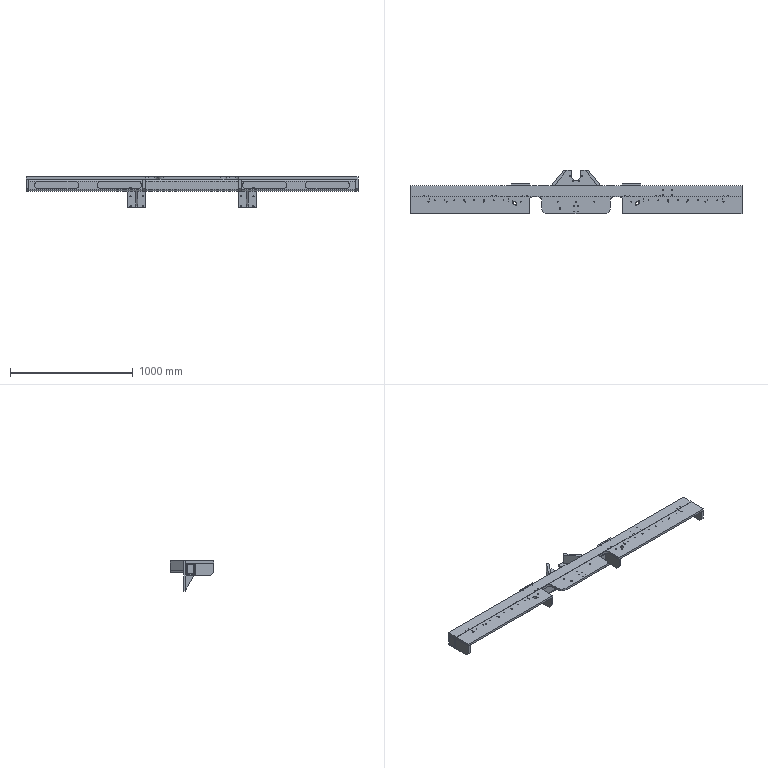Component | SolidWorks | LongSideMovingGuideRailBeam-Machined-1_LongSideMovingGuideRailBeam-Welded-0510-1 | 15 solids | 364 faces | volume 20520662 mm3 | cylinder 229 | plane 125 | cone 10 | commonest cylinder face diameters 8.5 x56 6 x42 6.8 x32 8 x26 5 x16 11 x8 6.6 x8 4.2 x8 | material Q235-A